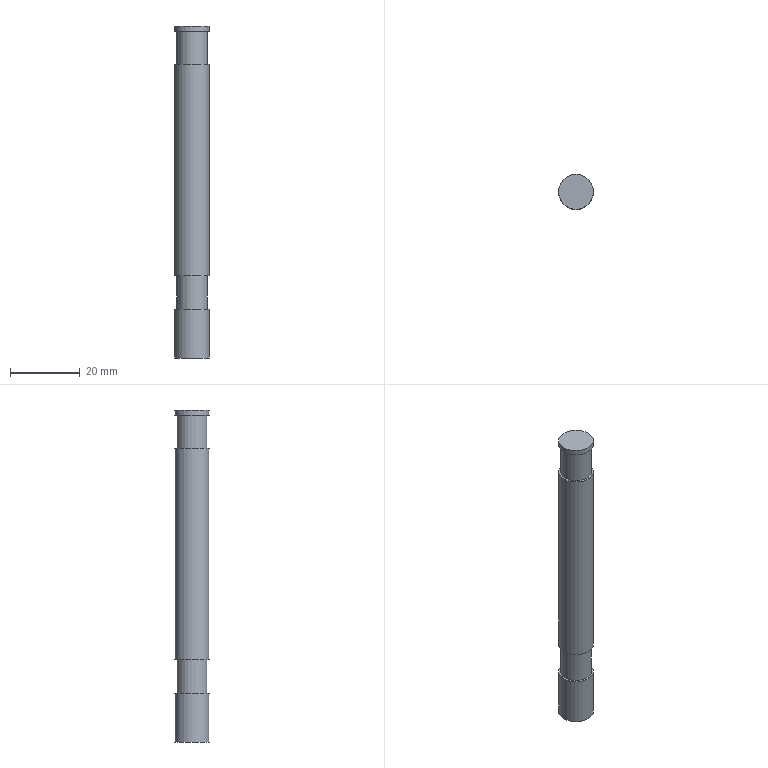Component | NX | FIXING_SCREW | 1 solid | 11 faces | box 10 x 10 x 95 mm | volume 7120 mm3 | plane 6 | cylinder 5 | commonest cylinder face diameters 10 x3 8.782 x2
STEP:
#1=CARTESIAN_POINT('',(0.,0.,0.));
#2=DIRECTION('',(0.,0.,1.));
#3=DIRECTION('',(1.,0.,0.));
#4=AXIS2_PLACEMENT_3D('',#1,#2,#3);
#5=CARTESIAN_POINT('',(5.,67.,21.5));
#6=VERTEX_POINT('',#5);
#7=CARTESIAN_POINT('',(0.,67.,21.5));
#8=DIRECTION('',(0.,0.,-1.));
#9=DIRECTION('',(1.,0.,0.));
#10=AXIS2_PLACEMENT_3D('',#7,#8,#9);
#11=CIRCLE('',#10,5.);
#12=CARTESIAN_POINT('',(0.,67.,-2.));
#13=DIRECTION('',(0.,0.,1.));
#14=DIRECTION('',(1.,0.,0.));
#15=AXIS2_PLACEMENT_3D('',#12,#13,#14);
#16=CYLINDRICAL_SURFACE('',#15,5.);
#17=CARTESIAN_POINT('',(6.283,23.5));
#18=DIRECTION('',(-1.,0.));
#19=VECTOR('',#18,1.);
#20=LINE('',#17,#19);
#21=(GEOMETRIC_REPRESENTATION_CONTEXT(2)PARAMETRIC_REPRESENTATION_CONTEXT()REPRESENTATION_CONTEXT('',''));
#22=DEFINITIONAL_REPRESENTATION('',(#20),#21);
#23=PCURVE('',#16,#22);
#24=CARTESIAN_POINT('',(0.,67.,21.5));
#25=DIRECTION('',(0.,0.,1.));
#26=DIRECTION('',(1.,0.,0.));
#27=AXIS2_PLACEMENT_3D('',#24,#25,#26);
#28=PLANE('',#27);
#29=CARTESIAN_POINT('',(5.,0.));
#30=CARTESIAN_POINT('',(5.,-8.66));
#31=CARTESIAN_POINT('',(-2.5,-4.33));
#32=CARTESIAN_POINT('',(-10.,-0.));
#33=CARTESIAN_POINT('',(-2.5,4.33));
#34=CARTESIAN_POINT('',(5.,8.66));
#35=CARTESIAN_POINT('',(5.,0.));
#36=(BOUNDED_CURVE()B_SPLINE_CURVE(2,(#29,#30,#31,#32,#33,#34,#35),.UNSPECIFIED.,.T.,.F.)B_SPLINE_CURVE_WITH_KNOTS((1,2,2,2,2,1),(-2.094,0.,2.094,4.189,6.283,8.378),.UNSPECIFIED.)CURVE()GEOMETRIC_REPRESENTATION_ITEM()RATIONAL_B_SPLINE_CURVE((1.,0.5,1.,0.5,1.,0.5,1.))REPRESENTATION_ITEM(''));
#37=(GEOMETRIC_REPRESENTATION_CONTEXT(2)PARAMETRIC_REPRESENTATION_CONTEXT()REPRESENTATION_CONTEXT('',''));
#38=DEFINITIONAL_REPRESENTATION('',(#36),#37);
#39=PCURVE('',#28,#38);
#40=SURFACE_CURVE('',#11,(#23,#39),.PCURVE_S1.);
#41=EDGE_CURVE('',#6,#6,#40,.T.);
#42=ORIENTED_EDGE('',*,*,#41,.F.);
#43=CARTESIAN_POINT('',(5.,67.,82.));
#44=VERTEX_POINT('',#43);
#45=CARTESIAN_POINT('',(5.,67.,21.5));
#46=CARTESIAN_POINT('',(5.,67.,82.));
#47=B_SPLINE_CURVE_WITH_KNOTS('',1,(#45,#46),.UNSPECIFIED.,.F.,.F.,(2,2),(23.5,84.),.PIECEWISE_BEZIER_KNOTS.);
#48=CARTESIAN_POINT('',(6.283,0.));
#49=DIRECTION('',(0.,1.));
#50=VECTOR('',#49,1.);
#51=LINE('',#48,#50);
#52=(GEOMETRIC_REPRESENTATION_CONTEXT(2)PARAMETRIC_REPRESENTATION_CONTEXT()REPRESENTATION_CONTEXT('',''));
#53=DEFINITIONAL_REPRESENTATION('',(#51),#52);
#54=PCURVE('',#16,#53);
#55=CARTESIAN_POINT('',(0.,0.));
#56=DIRECTION('',(0.,1.));
#57=VECTOR('',#56,1.);
#58=LINE('',#55,#57);
#59=(GEOMETRIC_REPRESENTATION_CONTEXT(2)PARAMETRIC_REPRESENTATION_CONTEXT()REPRESENTATION_CONTEXT('',''));
#60=DEFINITIONAL_REPRESENTATION('',(#58),#59);
#61=PCURVE('',#16,#60);
#62=SEAM_CURVE('',#47,(#54,#61),.PCURVE_S1.);
#63=EDGE_CURVE('',#6,#44,#62,.T.);
#64=ORIENTED_EDGE('',*,*,#63,.T.);
#65=CARTESIAN_POINT('',(0.,67.,82.));
#66=DIRECTION('',(0.,0.,-1.));
#67=DIRECTION('',(1.,0.,0.));
#68=AXIS2_PLACEMENT_3D('',#65,#66,#67);
#69=CIRCLE('',#68,5.);
#70=CARTESIAN_POINT('',(6.283,84.));
#71=DIRECTION('',(-1.,0.));
#72=VECTOR('',#71,1.);
#73=LINE('',#70,#72);
#74=(GEOMETRIC_REPRESENTATION_CONTEXT(2)PARAMETRIC_REPRESENTATION_CONTEXT()REPRESENTATION_CONTEXT('',''));
#75=DEFINITIONAL_REPRESENTATION('',(#73),#74);
#76=PCURVE('',#16,#75);
#77=CARTESIAN_POINT('',(0.,67.,82.));
#78=DIRECTION('',(0.,0.,1.));
#79=DIRECTION('',(1.,0.,0.));
#80=AXIS2_PLACEMENT_3D('',#77,#78,#79);
#81=PLANE('',#80);
#82=CARTESIAN_POINT('',(5.,0.));
#83=CARTESIAN_POINT('',(5.,-8.66));
#84=CARTESIAN_POINT('',(-2.5,-4.33));
#85=CARTESIAN_POINT('',(-10.,-0.));
#86=CARTESIAN_POINT('',(-2.5,4.33));
#87=CARTESIAN_POINT('',(5.,8.66));
#88=CARTESIAN_POINT('',(5.,0.));
#89=(BOUNDED_CURVE()B_SPLINE_CURVE(2,(#82,#83,#84,#85,#86,#87,#88),.UNSPECIFIED.,.T.,.F.)B_SPLINE_CURVE_WITH_KNOTS((1,2,2,2,2,1),(-2.094,0.,2.094,4.189,6.283,8.378),.UNSPECIFIED.)CURVE()GEOMETRIC_REPRESENTATION_ITEM()RATIONAL_B_SPLINE_CURVE((1.,0.5,1.,0.5,1.,0.5,1.))REPRESENTATION_ITEM(''));
#90=(GEOMETRIC_REPRESENTATION_CONTEXT(2)PARAMETRIC_REPRESENTATION_CONTEXT()REPRESENTATION_CONTEXT('',''));
#91=DEFINITIONAL_REPRESENTATION('',(#89),#90);
#92=PCURVE('',#81,#91);
#93=SURFACE_CURVE('',#69,(#76,#92),.PCURVE_S1.);
#94=EDGE_CURVE('',#44,#44,#93,.T.);
#95=ORIENTED_EDGE('',*,*,#94,.T.);
#96=ORIENTED_EDGE('',*,*,#63,.F.);
#97=EDGE_LOOP('',(#42,#64,#95,#96));
#98=FACE_BOUND('',#97,.T.);
#99=ADVANCED_FACE('',(#98),#16,.T.);
#100=CARTESIAN_POINT('',(4.391,67.,21.5));
#101=VERTEX_POINT('',#100);
#102=CARTESIAN_POINT('',(0.,67.,21.5));
#103=DIRECTION('',(0.,0.,-1.));
#104=DIRECTION('',(1.,0.,0.));
#105=AXIS2_PLACEMENT_3D('',#102,#103,#104);
#106=CIRCLE('',#105,4.391);
#107=CARTESIAN_POINT('',(0.,67.,21.5));
#108=DIRECTION('',(0.,0.,-1.));
#109=DIRECTION('',(-1.,0.,0.));
#110=AXIS2_PLACEMENT_3D('',#107,#108,#109);
#111=CYLINDRICAL_SURFACE('',#110,4.391);
#112=CARTESIAN_POINT('',(3.142,0.));
#113=DIRECTION('',(1.,0.));
#114=VECTOR('',#113,1.);
#115=LINE('',#112,#114);
#116=(GEOMETRIC_REPRESENTATION_CONTEXT(2)PARAMETRIC_REPRESENTATION_CONTEXT()REPRESENTATION_CONTEXT('',''));
#117=DEFINITIONAL_REPRESENTATION('',(#115),#116);
#118=PCURVE('',#111,#117);
#119=CARTESIAN_POINT('',(4.391,0.));
#120=CARTESIAN_POINT('',(4.391,-7.606));
#121=CARTESIAN_POINT('',(-2.196,-3.803));
#122=CARTESIAN_POINT('',(-8.782,-0.));
#123=CARTESIAN_POINT('',(-2.196,3.803));
#124=CARTESIAN_POINT('',(4.391,7.606));
#125=CARTESIAN_POINT('',(4.391,0.));
#126=(BOUNDED_CURVE()B_SPLINE_CURVE(2,(#119,#120,#121,#122,#123,#124,#125),.UNSPECIFIED.,.T.,.F.)B_SPLINE_CURVE_WITH_KNOTS((1,2,2,2,2,1),(-2.094,0.,2.094,4.189,6.283,8.378),.UNSPECIFIED.)CURVE()GEOMETRIC_REPRESENTATION_ITEM()RATIONAL_B_SPLINE_CURVE((1.,0.5,1.,0.5,1.,0.5,1.))REPRESENTATION_ITEM(''));
#127=(GEOMETRIC_REPRESENTATION_CONTEXT(2)PARAMETRIC_REPRESENTATION_CONTEXT()REPRESENTATION_CONTEXT('',''));
#128=DEFINITIONAL_REPRESENTATION('',(#126),#127);
#129=PCURVE('',#28,#128);
#130=SURFACE_CURVE('',#106,(#118,#129),.PCURVE_S1.);
#131=EDGE_CURVE('',#101,#101,#130,.T.);
#132=ORIENTED_EDGE('',*,*,#131,.T.);
#133=CARTESIAN_POINT('',(4.391,67.,12.));
#134=VERTEX_POINT('',#133);
#135=CARTESIAN_POINT('',(4.391,67.,21.5));
#136=CARTESIAN_POINT('',(4.391,67.,12.));
#137=B_SPLINE_CURVE_WITH_KNOTS('',1,(#135,#136),.UNSPECIFIED.,.F.,.F.,(2,2),(0.,9.5),.PIECEWISE_BEZIER_KNOTS.);
#138=CARTESIAN_POINT('',(9.425,0.));
#139=DIRECTION('',(0.,1.));
#140=VECTOR('',#139,1.);
#141=LINE('',#138,#140);
#142=(GEOMETRIC_REPRESENTATION_CONTEXT(2)PARAMETRIC_REPRESENTATION_CONTEXT()REPRESENTATION_CONTEXT('',''));
#143=DEFINITIONAL_REPRESENTATION('',(#141),#142);
#144=PCURVE('',#111,#143);
#145=CARTESIAN_POINT('',(3.142,0.));
#146=DIRECTION('',(0.,1.));
#147=VECTOR('',#146,1.);
#148=LINE('',#145,#147);
#149=(GEOMETRIC_REPRESENTATION_CONTEXT(2)PARAMETRIC_REPRESENTATION_CONTEXT()REPRESENTATION_CONTEXT('',''));
#150=DEFINITIONAL_REPRESENTATION('',(#148),#149);
#151=PCURVE('',#111,#150);
#152=SEAM_CURVE('',#137,(#144,#151),.PCURVE_S1.);
#153=EDGE_CURVE('',#101,#134,#152,.T.);
#154=ORIENTED_EDGE('',*,*,#153,.T.);
#155=CARTESIAN_POINT('',(0.,67.,12.));
#156=DIRECTION('',(0.,0.,-1.));
#157=DIRECTION('',(1.,0.,0.));
#158=AXIS2_PLACEMENT_3D('',#155,#156,#157);
#159=CIRCLE('',#158,4.391);
#160=CARTESIAN_POINT('',(3.142,9.5));
#161=DIRECTION('',(1.,0.));
#162=VECTOR('',#161,1.);
#163=LINE('',#160,#162);
#164=(GEOMETRIC_REPRESENTATION_CONTEXT(2)PARAMETRIC_REPRESENTATION_CONTEXT()REPRESENTATION_CONTEXT('',''));
#165=DEFINITIONAL_REPRESENTATION('',(#163),#164);
#166=PCURVE('',#111,#165);
#167=CARTESIAN_POINT('',(0.,67.,12.));
#168=DIRECTION('',(0.,0.,1.));
#169=DIRECTION('',(1.,0.,0.));
#170=AXIS2_PLACEMENT_3D('',#167,#168,#169);
#171=PLANE('',#170);
#172=CARTESIAN_POINT('',(4.391,0.));
#173=CARTESIAN_POINT('',(4.391,-7.606));
#174=CARTESIAN_POINT('',(-2.196,-3.803));
#175=CARTESIAN_POINT('',(-8.782,-0.));
#176=CARTESIAN_POINT('',(-2.196,3.803));
#177=CARTESIAN_POINT('',(4.391,7.606));
#178=CARTESIAN_POINT('',(4.391,0.));
#179=(BOUNDED_CURVE()B_SPLINE_CURVE(2,(#172,#173,#174,#175,#176,#177,#178),.UNSPECIFIED.,.T.,.F.)B_SPLINE_CURVE_WITH_KNOTS((1,2,2,2,2,1),(-2.094,0.,2.094,4.189,6.283,8.378),.UNSPECIFIED.)CURVE()GEOMETRIC_REPRESENTATION_ITEM()RATIONAL_B_SPLINE_CURVE((1.,0.5,1.,0.5,1.,0.5,1.))REPRESENTATION_ITEM(''));
#180=(GEOMETRIC_REPRESENTATION_CONTEXT(2)PARAMETRIC_REPRESENTATION_CONTEXT()REPRESENTATION_CONTEXT('',''));
#181=DEFINITIONAL_REPRESENTATION('',(#179),#180);
#182=PCURVE('',#171,#181);
#183=SURFACE_CURVE('',#159,(#166,#182),.PCURVE_S1.);
#184=EDGE_CURVE('',#134,#134,#183,.T.);
#185=ORIENTED_EDGE('',*,*,#184,.F.);
#186=ORIENTED_EDGE('',*,*,#153,.F.);
#187=EDGE_LOOP('',(#132,#154,#185,#186));
#188=FACE_BOUND('',#187,.T.);
#189=ADVANCED_FACE('',(#188),#111,.T.);
#190=ORIENTED_EDGE('',*,*,#41,.T.);
#191=EDGE_LOOP('',(#190));
#192=FACE_BOUND('',#191,.T.);
#193=ORIENTED_EDGE('',*,*,#131,.F.);
#194=EDGE_LOOP('',(#193));
#195=FACE_BOUND('',#194,.T.);
#196=ADVANCED_FACE('',(#192,#195),#28,.F.);
#197=CARTESIAN_POINT('',(5.,67.,12.));
#198=VERTEX_POINT('',#197);
#199=CARTESIAN_POINT('',(0.,67.,12.));
#200=DIRECTION('',(0.,0.,-1.));
#201=DIRECTION('',(1.,0.,0.));
#202=AXIS2_PLACEMENT_3D('',#199,#200,#201);
#203=CIRCLE('',#202,5.);
#204=CARTESIAN_POINT('',(5.,0.));
#205=CARTESIAN_POINT('',(5.,-8.66));
#206=CARTESIAN_POINT('',(-2.5,-4.33));
#207=CARTESIAN_POINT('',(-10.,-0.));
#208=CARTESIAN_POINT('',(-2.5,4.33));
#209=CARTESIAN_POINT('',(5.,8.66));
#210=CARTESIAN_POINT('',(5.,0.));
#211=(BOUNDED_CURVE()B_SPLINE_CURVE(2,(#204,#205,#206,#207,#208,#209,#210),.UNSPECIFIED.,.T.,.F.)B_SPLINE_CURVE_WITH_KNOTS((1,2,2,2,2,1),(-2.094,0.,2.094,4.189,6.283,8.378),.UNSPECIFIED.)CURVE()GEOMETRIC_REPRESENTATION_ITEM()RATIONAL_B_SPLINE_CURVE((1.,0.5,1.,0.5,1.,0.5,1.))REPRESENTATION_ITEM(''));
#212=(GEOMETRIC_REPRESENTATION_CONTEXT(2)PARAMETRIC_REPRESENTATION_CONTEXT()REPRESENTATION_CONTEXT('',''));
#213=DEFINITIONAL_REPRESENTATION('',(#211),#212);
#214=PCURVE('',#171,#213);
#215=CARTESIAN_POINT('',(0.,67.,-2.));
#216=DIRECTION('',(0.,0.,1.));
#217=DIRECTION('',(1.,0.,0.));
#218=AXIS2_PLACEMENT_3D('',#215,#216,#217);
#219=CYLINDRICAL_SURFACE('',#218,5.);
#220=CARTESIAN_POINT('',(6.283,14.));
#221=DIRECTION('',(-1.,0.));
#222=VECTOR('',#221,1.);
#223=LINE('',#220,#222);
#224=(GEOMETRIC_REPRESENTATION_CONTEXT(2)PARAMETRIC_REPRESENTATION_CONTEXT()REPRESENTATION_CONTEXT('',''));
#225=DEFINITIONAL_REPRESENTATION('',(#223),#224);
#226=PCURVE('',#219,#225);
#227=SURFACE_CURVE('',#203,(#214,#226),.PCURVE_S1.);
#228=EDGE_CURVE('',#198,#198,#227,.T.);
#229=ORIENTED_EDGE('',*,*,#228,.F.);
#230=EDGE_LOOP('',(#229));
#231=FACE_BOUND('',#230,.T.);
#232=ORIENTED_EDGE('',*,*,#184,.T.);
#233=EDGE_LOOP('',(#232));
#234=FACE_BOUND('',#233,.T.);
#235=ADVANCED_FACE('',(#231,#234),#171,.T.);
#236=CARTESIAN_POINT('',(5.,67.,-2.));
#237=VERTEX_POINT('',#236);
#238=CARTESIAN_POINT('',(0.,67.,-2.));
#239=DIRECTION('',(0.,0.,1.));
#240=DIRECTION('',(1.,0.,0.));
#241=AXIS2_PLACEMENT_3D('',#238,#239,#240);
#242=CIRCLE('',#241,5.);
#243=CARTESIAN_POINT('',(0.,67.,-2.));
#244=DIRECTION('',(0.,0.,-1.));
#245=DIRECTION('',(-1.,0.,0.));
#246=AXIS2_PLACEMENT_3D('',#243,#244,#245);
#247=PLANE('',#246);
#248=CARTESIAN_POINT('',(-5.,0.));
#249=CARTESIAN_POINT('',(-5.,8.66));
#250=CARTESIAN_POINT('',(2.5,4.33));
#251=CARTESIAN_POINT('',(10.,0.));
#252=CARTESIAN_POINT('',(2.5,-4.33));
#253=CARTESIAN_POINT('',(-5.,-8.66));
#254=CARTESIAN_POINT('',(-5.,0.));
#255=(BOUNDED_CURVE()B_SPLINE_CURVE(2,(#248,#249,#250,#251,#252,#253,#254),.UNSPECIFIED.,.T.,.F.)B_SPLINE_CURVE_WITH_KNOTS((1,2,2,2,2,1),(-2.094,0.,2.094,4.189,6.283,8.378),.UNSPECIFIED.)CURVE()GEOMETRIC_REPRESENTATION_ITEM()RATIONAL_B_SPLINE_CURVE((1.,0.5,1.,0.5,1.,0.5,1.))REPRESENTATION_ITEM(''));
#256=(GEOMETRIC_REPRESENTATION_CONTEXT(2)PARAMETRIC_REPRESENTATION_CONTEXT()REPRESENTATION_CONTEXT('',''));
#257=DEFINITIONAL_REPRESENTATION('',(#255),#256);
#258=PCURVE('',#247,#257);
#259=CARTESIAN_POINT('',(0.,0.));
#260=DIRECTION('',(1.,0.));
#261=VECTOR('',#260,1.);
#262=LINE('',#259,#261);
#263=(GEOMETRIC_REPRESENTATION_CONTEXT(2)PARAMETRIC_REPRESENTATION_CONTEXT()REPRESENTATION_CONTEXT('',''));
#264=DEFINITIONAL_REPRESENTATION('',(#262),#263);
#265=PCURVE('',#219,#264);
#266=SURFACE_CURVE('',#242,(#258,#265),.PCURVE_S1.);
#267=EDGE_CURVE('',#237,#237,#266,.T.);
#268=ORIENTED_EDGE('',*,*,#267,.F.);
#269=EDGE_LOOP('',(#268));
#270=FACE_BOUND('',#269,.T.);
#271=ADVANCED_FACE('',(#270),#247,.T.);
#272=ORIENTED_EDGE('',*,*,#267,.T.);
#273=CARTESIAN_POINT('',(5.,67.,-2.));
#274=CARTESIAN_POINT('',(5.,67.,12.));
#275=B_SPLINE_CURVE_WITH_KNOTS('',1,(#273,#274),.UNSPECIFIED.,.F.,.F.,(2,2),(0.,14.),.PIECEWISE_BEZIER_KNOTS.);
#276=CARTESIAN_POINT('',(6.283,0.));
#277=DIRECTION('',(0.,1.));
#278=VECTOR('',#277,1.);
#279=LINE('',#276,#278);
#280=(GEOMETRIC_REPRESENTATION_CONTEXT(2)PARAMETRIC_REPRESENTATION_CONTEXT()REPRESENTATION_CONTEXT('',''));
#281=DEFINITIONAL_REPRESENTATION('',(#279),#280);
#282=PCURVE('',#219,#281);
#283=CARTESIAN_POINT('',(0.,0.));
#284=DIRECTION('',(0.,1.));
#285=VECTOR('',#284,1.);
#286=LINE('',#283,#285);
#287=(GEOMETRIC_REPRESENTATION_CONTEXT(2)PARAMETRIC_REPRESENTATION_CONTEXT()REPRESENTATION_CONTEXT('',''));
#288=DEFINITIONAL_REPRESENTATION('',(#286),#287);
#289=PCURVE('',#219,#288);
#290=SEAM_CURVE('',#275,(#282,#289),.PCURVE_S1.);
#291=EDGE_CURVE('',#237,#198,#290,.T.);
#292=ORIENTED_EDGE('',*,*,#291,.T.);
#293=ORIENTED_EDGE('',*,*,#228,.T.);
#294=ORIENTED_EDGE('',*,*,#291,.F.);
#295=EDGE_LOOP('',(#272,#292,#293,#294));
#296=FACE_BOUND('',#295,.T.);
#297=ADVANCED_FACE('',(#296),#219,.T.);
#298=CARTESIAN_POINT('',(4.391,67.,91.5));
#299=VERTEX_POINT('',#298);
#300=CARTESIAN_POINT('',(0.,67.,91.5));
#301=DIRECTION('',(0.,0.,-1.));
#302=DIRECTION('',(1.,0.,0.));
#303=AXIS2_PLACEMENT_3D('',#300,#301,#302);
#304=CIRCLE('',#303,4.391);
#305=CARTESIAN_POINT('',(0.,67.,91.5));
#306=DIRECTION('',(0.,0.,-1.));
#307=DIRECTION('',(-1.,0.,0.));
#308=AXIS2_PLACEMENT_3D('',#305,#306,#307);
#309=CYLINDRICAL_SURFACE('',#308,4.391);
#310=CARTESIAN_POINT('',(3.142,0.));
#311=DIRECTION('',(1.,0.));
#312=VECTOR('',#311,1.);
#313=LINE('',#310,#312);
#314=(GEOMETRIC_REPRESENTATION_CONTEXT(2)PARAMETRIC_REPRESENTATION_CONTEXT()REPRESENTATION_CONTEXT('',''));
#315=DEFINITIONAL_REPRESENTATION('',(#313),#314);
#316=PCURVE('',#309,#315);
#317=CARTESIAN_POINT('',(0.,67.,91.5));
#318=DIRECTION('',(0.,0.,1.));
#319=DIRECTION('',(1.,0.,0.));
#320=AXIS2_PLACEMENT_3D('',#317,#318,#319);
#321=PLANE('',#320);
#322=CARTESIAN_POINT('',(4.391,0.));
#323=CARTESIAN_POINT('',(4.391,-7.606));
#324=CARTESIAN_POINT('',(-2.196,-3.803));
#325=CARTESIAN_POINT('',(-8.782,-0.));
#326=CARTESIAN_POINT('',(-2.196,3.803));
#327=CARTESIAN_POINT('',(4.391,7.606));
#328=CARTESIAN_POINT('',(4.391,0.));
#329=(BOUNDED_CURVE()B_SPLINE_CURVE(2,(#322,#323,#324,#325,#326,#327,#328),.UNSPECIFIED.,.T.,.F.)B_SPLINE_CURVE_WITH_KNOTS((1,2,2,2,2,1),(-2.094,0.,2.094,4.189,6.283,8.378),.UNSPECIFIED.)CURVE()GEOMETRIC_REPRESENTATION_ITEM()RATIONAL_B_SPLINE_CURVE((1.,0.5,1.,0.5,1.,0.5,1.))REPRESENTATION_ITEM(''));
#330=(GEOMETRIC_REPRESENTATION_CONTEXT(2)PARAMETRIC_REPRESENTATION_CONTEXT()REPRESENTATION_CONTEXT('',''));
#331=DEFINITIONAL_REPRESENTATION('',(#329),#330);
#332=PCURVE('',#321,#331);
#333=SURFACE_CURVE('',#304,(#316,#332),.PCURVE_S1.);
#334=EDGE_CURVE('',#299,#299,#333,.T.);
#335=ORIENTED_EDGE('',*,*,#334,.T.);
#336=CARTESIAN_POINT('',(4.391,67.,82.));
#337=VERTEX_POINT('',#336);
#338=CARTESIAN_POINT('',(4.391,67.,91.5));
#339=CARTESIAN_POINT('',(4.391,67.,82.));
#340=B_SPLINE_CURVE_WITH_KNOTS('',1,(#338,#339),.UNSPECIFIED.,.F.,.F.,(2,2),(0.,9.5),.PIECEWISE_BEZIER_KNOTS.);
#341=CARTESIAN_POINT('',(9.425,0.));
#342=DIRECTION('',(0.,1.));
#343=VECTOR('',#342,1.);
#344=LINE('',#341,#343);
#345=(GEOMETRIC_REPRESENTATION_CONTEXT(2)PARAMETRIC_REPRESENTATION_CONTEXT()REPRESENTATION_CONTEXT('',''));
#346=DEFINITIONAL_REPRESENTATION('',(#344),#345);
#347=PCURVE('',#309,#346);
#348=CARTESIAN_POINT('',(3.142,0.));
#349=DIRECTION('',(0.,1.));
#350=VECTOR('',#349,1.);
#351=LINE('',#348,#350);
#352=(GEOMETRIC_REPRESENTATION_CONTEXT(2)PARAMETRIC_REPRESENTATION_CONTEXT()REPRESENTATION_CONTEXT('',''));
#353=DEFINITIONAL_REPRESENTATION('',(#351),#352);
#354=PCURVE('',#309,#353);
#355=SEAM_CURVE('',#340,(#347,#354),.PCURVE_S1.);
#356=EDGE_CURVE('',#299,#337,#355,.T.);
#357=ORIENTED_EDGE('',*,*,#356,.T.);
#358=CARTESIAN_POINT('',(0.,67.,82.));
#359=DIRECTION('',(0.,0.,-1.));
#360=DIRECTION('',(1.,0.,0.));
#361=AXIS2_PLACEMENT_3D('',#358,#359,#360);
#362=CIRCLE('',#361,4.391);
#363=CARTESIAN_POINT('',(3.142,9.5));
#364=DIRECTION('',(1.,0.));
#365=VECTOR('',#364,1.);
#366=LINE('',#363,#365);
#367=(GEOMETRIC_REPRESENTATION_CONTEXT(2)PARAMETRIC_REPRESENTATION_CONTEXT()REPRESENTATION_CONTEXT('',''));
#368=DEFINITIONAL_REPRESENTATION('',(#366),#367);
#369=PCURVE('',#309,#368);
#370=CARTESIAN_POINT('',(4.391,0.));
#371=CARTESIAN_POINT('',(4.391,-7.606));
#372=CARTESIAN_POINT('',(-2.196,-3.803));
#373=CARTESIAN_POINT('',(-8.782,-0.));
#374=CARTESIAN_POINT('',(-2.196,3.803));
#375=CARTESIAN_POINT('',(4.391,7.606));
#376=CARTESIAN_POINT('',(4.391,0.));
#377=(BOUNDED_CURVE()B_SPLINE_CURVE(2,(#370,#371,#372,#373,#374,#375,#376),.UNSPECIFIED.,.T.,.F.)B_SPLINE_CURVE_WITH_KNOTS((1,2,2,2,2,1),(-2.094,0.,2.094,4.189,6.283,8.378),.UNSPECIFIED.)CURVE()GEOMETRIC_REPRESENTATION_ITEM()RATIONAL_B_SPLINE_CURVE((1.,0.5,1.,0.5,1.,0.5,1.))REPRESENTATION_ITEM(''));
#378=(GEOMETRIC_REPRESENTATION_CONTEXT(2)PARAMETRIC_REPRESENTATION_CONTEXT()REPRESENTATION_CONTEXT('',''));
#379=DEFINITIONAL_REPRESENTATION('',(#377),#378);
#380=PCURVE('',#81,#379);
#381=SURFACE_CURVE('',#362,(#369,#380),.PCURVE_S1.);
#382=EDGE_CURVE('',#337,#337,#381,.T.);
#383=ORIENTED_EDGE('',*,*,#382,.F.);
#384=ORIENTED_EDGE('',*,*,#356,.F.);
#385=EDGE_LOOP('',(#335,#357,#383,#384));
#386=FACE_BOUND('',#385,.T.);
#387=ADVANCED_FACE('',(#386),#309,.T.);
#388=CARTESIAN_POINT('',(5.,67.,91.5));
#389=VERTEX_POINT('',#388);
#390=CARTESIAN_POINT('',(0.,67.,91.5));
#391=DIRECTION('',(0.,0.,-1.));
#392=DIRECTION('',(1.,0.,0.));
#393=AXIS2_PLACEMENT_3D('',#390,#391,#392);
#394=CIRCLE('',#393,5.);
#395=CARTESIAN_POINT('',(5.,0.));
#396=CARTESIAN_POINT('',(5.,-8.66));
#397=CARTESIAN_POINT('',(-2.5,-4.33));
#398=CARTESIAN_POINT('',(-10.,-0.));
#399=CARTESIAN_POINT('',(-2.5,4.33));
#400=CARTESIAN_POINT('',(5.,8.66));
#401=CARTESIAN_POINT('',(5.,0.));
#402=(BOUNDED_CURVE()B_SPLINE_CURVE(2,(#395,#396,#397,#398,#399,#400,#401),.UNSPECIFIED.,.T.,.F.)B_SPLINE_CURVE_WITH_KNOTS((1,2,2,2,2,1),(-2.094,0.,2.094,4.189,6.283,8.378),.UNSPECIFIED.)CURVE()GEOMETRIC_REPRESENTATION_ITEM()RATIONAL_B_SPLINE_CURVE((1.,0.5,1.,0.5,1.,0.5,1.))REPRESENTATION_ITEM(''));
#403=(GEOMETRIC_REPRESENTATION_CONTEXT(2)PARAMETRIC_REPRESENTATION_CONTEXT()REPRESENTATION_CONTEXT('',''));
#404=DEFINITIONAL_REPRESENTATION('',(#402),#403);
#405=PCURVE('',#321,#404);
#406=CARTESIAN_POINT('',(0.,67.,-2.));
#407=DIRECTION('',(0.,0.,1.));
#408=DIRECTION('',(1.,0.,0.));
#409=AXIS2_PLACEMENT_3D('',#406,#407,#408);
#410=CYLINDRICAL_SURFACE('',#409,5.);
#411=CARTESIAN_POINT('',(6.283,93.5));
#412=DIRECTION('',(-1.,0.));
#413=VECTOR('',#412,1.);
#414=LINE('',#411,#413);
#415=(GEOMETRIC_REPRESENTATION_CONTEXT(2)PARAMETRIC_REPRESENTATION_CONTEXT()REPRESENTATION_CONTEXT('',''));
#416=DEFINITIONAL_REPRESENTATION('',(#414),#415);
#417=PCURVE('',#410,#416);
#418=SURFACE_CURVE('',#394,(#405,#417),.PCURVE_S1.);
#419=EDGE_CURVE('',#389,#389,#418,.T.);
#420=ORIENTED_EDGE('',*,*,#419,.T.);
#421=EDGE_LOOP('',(#420));
#422=FACE_BOUND('',#421,.T.);
#423=ORIENTED_EDGE('',*,*,#334,.F.);
#424=EDGE_LOOP('',(#423));
#425=FACE_BOUND('',#424,.T.);
#426=ADVANCED_FACE('',(#422,#425),#321,.F.);
#427=ORIENTED_EDGE('',*,*,#94,.F.);
#428=EDGE_LOOP('',(#427));
#429=FACE_BOUND('',#428,.T.);
#430=ORIENTED_EDGE('',*,*,#382,.T.);
#431=EDGE_LOOP('',(#430));
#432=FACE_BOUND('',#431,.T.);
#433=ADVANCED_FACE('',(#429,#432),#81,.T.);
#434=CARTESIAN_POINT('',(5.,67.,93.));
#435=VERTEX_POINT('',#434);
#436=CARTESIAN_POINT('',(0.,67.,93.));
#437=DIRECTION('',(0.,0.,-1.));
#438=DIRECTION('',(1.,0.,0.));
#439=AXIS2_PLACEMENT_3D('',#436,#437,#438);
#440=CIRCLE('',#439,5.);
#441=CARTESIAN_POINT('',(0.,67.,93.));
#442=DIRECTION('',(0.,0.,1.));
#443=DIRECTION('',(1.,0.,0.));
#444=AXIS2_PLACEMENT_3D('',#441,#442,#443);
#445=PLANE('',#444);
#446=CARTESIAN_POINT('',(5.,0.));
#447=CARTESIAN_POINT('',(5.,-8.66));
#448=CARTESIAN_POINT('',(-2.5,-4.33));
#449=CARTESIAN_POINT('',(-10.,-0.));
#450=CARTESIAN_POINT('',(-2.5,4.33));
#451=CARTESIAN_POINT('',(5.,8.66));
#452=CARTESIAN_POINT('',(5.,0.));
#453=(BOUNDED_CURVE()B_SPLINE_CURVE(2,(#446,#447,#448,#449,#450,#451,#452),.UNSPECIFIED.,.T.,.F.)B_SPLINE_CURVE_WITH_KNOTS((1,2,2,2,2,1),(-2.094,0.,2.094,4.189,6.283,8.378),.UNSPECIFIED.)CURVE()GEOMETRIC_REPRESENTATION_ITEM()RATIONAL_B_SPLINE_CURVE((1.,0.5,1.,0.5,1.,0.5,1.))REPRESENTATION_ITEM(''));
#454=(GEOMETRIC_REPRESENTATION_CONTEXT(2)PARAMETRIC_REPRESENTATION_CONTEXT()REPRESENTATION_CONTEXT('',''));
#455=DEFINITIONAL_REPRESENTATION('',(#453),#454);
#456=PCURVE('',#445,#455);
#457=CARTESIAN_POINT('',(6.283,95.));
#458=DIRECTION('',(-1.,0.));
#459=VECTOR('',#458,1.);
#460=LINE('',#457,#459);
#461=(GEOMETRIC_REPRESENTATION_CONTEXT(2)PARAMETRIC_REPRESENTATION_CONTEXT()REPRESENTATION_CONTEXT('',''));
#462=DEFINITIONAL_REPRESENTATION('',(#460),#461);
#463=PCURVE('',#410,#462);
#464=SURFACE_CURVE('',#440,(#456,#463),.PCURVE_S1.);
#465=EDGE_CURVE('',#435,#435,#464,.T.);
#466=ORIENTED_EDGE('',*,*,#465,.F.);
#467=EDGE_LOOP('',(#466));
#468=FACE_BOUND('',#467,.T.);
#469=ADVANCED_FACE('',(#468),#445,.T.);
#470=ORIENTED_EDGE('',*,*,#419,.F.);
#471=CARTESIAN_POINT('',(5.,67.,91.5));
#472=CARTESIAN_POINT('',(5.,67.,93.));
#473=B_SPLINE_CURVE_WITH_KNOTS('',1,(#471,#472),.UNSPECIFIED.,.F.,.F.,(2,2),(93.5,95.),.PIECEWISE_BEZIER_KNOTS.);
#474=CARTESIAN_POINT('',(6.283,0.));
#475=DIRECTION('',(0.,1.));
#476=VECTOR('',#475,1.);
#477=LINE('',#474,#476);
#478=(GEOMETRIC_REPRESENTATION_CONTEXT(2)PARAMETRIC_REPRESENTATION_CONTEXT()REPRESENTATION_CONTEXT('',''));
#479=DEFINITIONAL_REPRESENTATION('',(#477),#478);
#480=PCURVE('',#410,#479);
#481=CARTESIAN_POINT('',(0.,0.));
#482=DIRECTION('',(0.,1.));
#483=VECTOR('',#482,1.);
#484=LINE('',#481,#483);
#485=(GEOMETRIC_REPRESENTATION_CONTEXT(2)PARAMETRIC_REPRESENTATION_CONTEXT()REPRESENTATION_CONTEXT('',''));
#486=DEFINITIONAL_REPRESENTATION('',(#484),#485);
#487=PCURVE('',#410,#486);
#488=SEAM_CURVE('',#473,(#480,#487),.PCURVE_S1.);
#489=EDGE_CURVE('',#389,#435,#488,.T.);
#490=ORIENTED_EDGE('',*,*,#489,.T.);
#491=ORIENTED_EDGE('',*,*,#465,.T.);
#492=ORIENTED_EDGE('',*,*,#489,.F.);
#493=EDGE_LOOP('',(#470,#490,#491,#492));
#494=FACE_BOUND('',#493,.T.);
#495=ADVANCED_FACE('',(#494),#410,.T.);
#496=CLOSED_SHELL('',(#99,#189,#196,#235,#271,#297,#387,#426,#433,#469,#495));
#497=MANIFOLD_SOLID_BREP('',#496);
#498=(LENGTH_UNIT()NAMED_UNIT(*)SI_UNIT(.MILLI.,.METRE.));
#499=UNCERTAINTY_MEASURE_WITH_UNIT(LENGTH_MEASURE(0.00001),#498,'','');
#500=(NAMED_UNIT(*)PLANE_ANGLE_UNIT()SI_UNIT($,.RADIAN.));
#501=(NAMED_UNIT(*)SI_UNIT($,.STERADIAN.)SOLID_ANGLE_UNIT());
#502=(GEOMETRIC_REPRESENTATION_CONTEXT(3)GLOBAL_UNCERTAINTY_ASSIGNED_CONTEXT((#499))GLOBAL_UNIT_ASSIGNED_CONTEXT((#498,#500,#501))REPRESENTATION_CONTEXT('',''));
#503=ADVANCED_BREP_SHAPE_REPRESENTATION('',(#4,#497),#502);